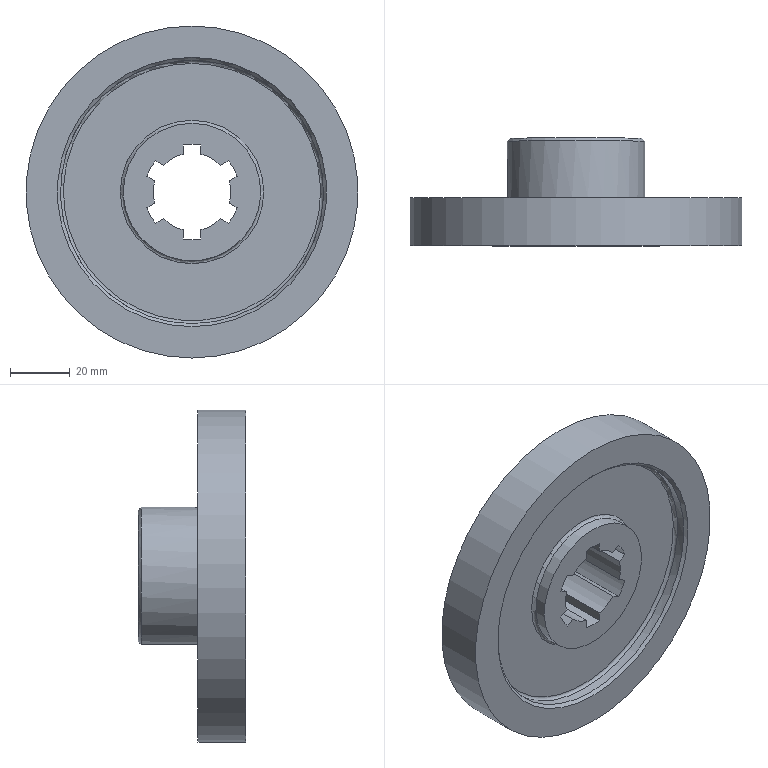Component | NX | ZHOU9-CHULUN2 | 1 solid | 37 faces | volume 142817 mm3 | plane 17 | cylinder 16 | torus 2 | cone 2 | commonest cylinder face diameters 26 x6 32 x6 46 x2 111 x1 88 x1